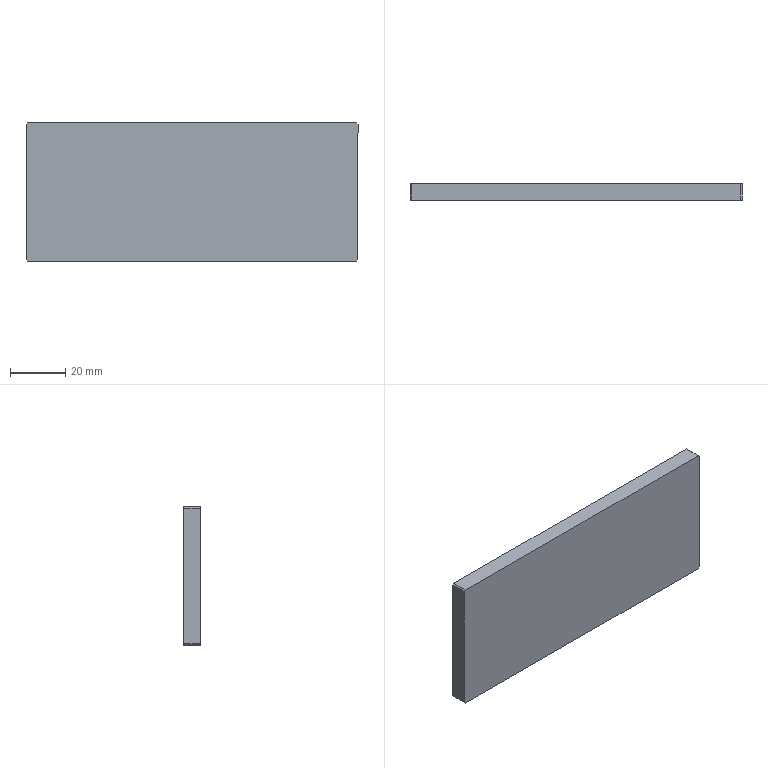Component | SolidWorks | 021-1 | 1 solid | 10 faces | box 120 x 6 x 50 mm | volume 35997 mm3 | plane 10 | material AL6061
build123d program:
from build123d import *

# Parameters (mm, degrees)
SKETCH1_W           = 50
SKETCH1_H           = 120
BOSS_EXTRUDE1_DEPTH = 6
CHAMFER1_SIZE       = 0.5


with BuildPart() as part:
    # Sketch1 → Boss-Extrude1 (new body)
    with BuildSketch(Plane.XY):
        Rectangle(SKETCH1_W, SKETCH1_H)
    extrude(amount=BOSS_EXTRUDE1_DEPTH)

    # Chamfer1
    chamfer1_edges = [part.edges().sort_by_distance(p)[0] for p in [
        (25, -60, 3),
        (-25, -60, 3),
        (-25, 60, 3),
        (25, 60, 3),
    ]]
    chamfer(chamfer1_edges, length=CHAMFER1_SIZE)


solid = part.part

# Placed as in the assembly
solid = solid.moved(Location((-240.455, -105.942, -154.304), (90, 0, 90)))